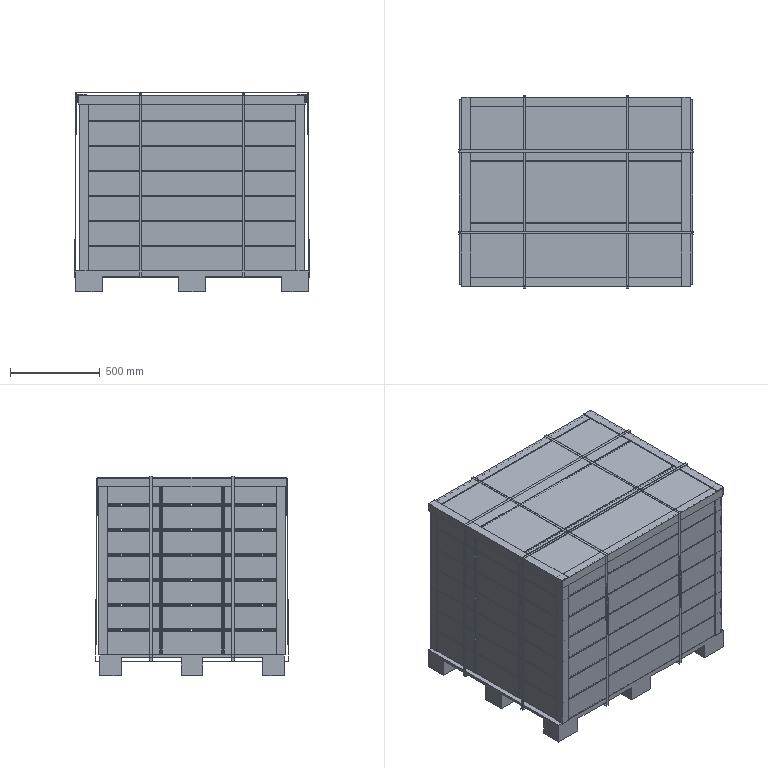Assembly | NX | mm | 34 component files | 34 solids | 431 faces | box 1307.7 x 1076.11 x 1110.92 mm | volume 176453760 mm3 | plane 419 | cylinder 12 | commonest cylinder face diameters 10 x6 6 x6
Bill of materials:
unnamed part 1 | 1 |  | Flat rectangular deck plate supported underneath by a 3x3 grid of rectangular blocks, which leaves open gaps between the blocks along both horizontal directions; the overall form resembles a pallet.
unnamed part 2 | 4 |  | Straight length of angle profile (L-shaped cross-section) with two legs that look roughly equal, cut square at both ends.
unnamed part 3 | 2 |  | Thin flat rectangular plate or sheet with no visible holes or other features; it is wider than it is tall in its main face view.
unnamed part 4 | 21 |  | Solid rectangular block or bar (a cuboid) with flat faces and sharp edges, and no visible features.
unnamed part 5 | 2 |  | Long straight angle profile (L-shaped cross-section) with legs that look roughly equal and square-cut ends, oriented horizontally.
unnamed part 6 | 2 |  | Long straight angle profile (L-shaped cross-section) with legs that look roughly equal and square-cut ends; it has the same form as the other horizontal angle but is shown in a mirrored or rotated orientation.
unnamed part 7 | 2 |  | Thin flat rectangular plate or sheet with no visible features; its face is close to square, a little taller than wide in its main face view.
Mates:
1. fix | carton 21 component
2. fix | assembly component
3. bond | carton 21 component | assembly component
4. bond | carton 20 component | assembly component
5. linear | assembly datumaxis | assembly cartesiancoordinatesystem | assembly cartesiancoordinatesystem | assembly cartesiancoordinatesystem
6. touch align | vertical_corner_protector 4 face | carton 1 face
7. touch align | vertical_corner_protector 4 face | carton 1 face
8. touch align | vertical_corner_protector 4 face | carton 20 face
9. touch align | vertical_corner_protector 3 face | carton 6 face
10. touch align | vertical_corner_protector 3 face | carton 6 face
11. touch align | vertical_corner_protector 3 face | carton 19 face
12. touch align | vertical_corner_protector 2 face | carton 6 face
13. touch align | vertical_corner_protector 2 face | carton 6 face
14. touch align | vertical_corner_protector 2 face | 103x135x10_pallet 1 face
15. touch align | vertical_corner_protector 1 face | carton 1 face
16. touch align | vertical_corner_protector 1 face | carton 1 face
17. touch align | vertical_corner_protector 1 face | 103x135x10_pallet 1 face
18. touch align | length_corner_protector 2 face | vertical_corner_protector 2 face
19. touch align | length_corner_protector 2 face | vertical_corner_protector 2 face
20. touch align | length_corner_protector 2 face | vertical_corner_protector 2 face
21. touch align | length_corner_protector 1 face | vertical_corner_protector 4 face
22. touch align | length_corner_protector 1 face | vertical_corner_protector 4 face
23. touch align | length_corner_protector 1 face | vertical_corner_protector 4 face
24. touch align | width_corner_protector 2 face | length_corner_protector 1 face
25. touch align | width_corner_protector 2 face | length_corner_protector 1 face
26. touch align | width_corner_protector 1 face | length_corner_protector 2 face
27. touch align | width_corner_protector 1 face | length_corner_protector 2 face
28. fix | assembly component
29. bond | short_packaging_strap 2 component | assembly component
30. bond | short_packaging_strap 1 component | assembly component
31. linear | assembly datumaxis | assembly cartesiancoordinatesystem | assembly cartesiancoordinatesystem
32. fix | assembly component
33. bond | long_packaging_strap 2 component | assembly component
34. bond | long_packaging_strap 1 component | assembly component
35. linear | assembly datumaxis | assembly cartesiancoordinatesystem | assembly cartesiancoordinatesystem
36. bond | carton 19 component | assembly component
37. fix | assembly component
38. bond | carton 19 component | assembly component
39. bond | carton 21 component | assembly component
40. bond | carton 20 component | assembly component
41. bond | carton 18 component | assembly component
42. bond | carton 17 component | assembly component
43. bond | carton 16 component | assembly component
44. linear | assembly datumaxis | assembly cartesiancoordinatesystem | assembly cartesiancoordinatesystem | assembly cartesiancoordinatesystem | assembly cartesiancoordinatesystem | assembly cartesiancoordinatesystem | assembly cartesiancoordinatesystem | assembly cartesiancoordinatesystem
45. linear | assembly datumaxis | assembly cartesiancoordinatesystem | assembly cartesiancoordinatesystem | assembly cartesiancoordinatesystem | assembly cartesiancoordinatesystem | assembly cartesiancoordinatesystem | assembly cartesiancoordinatesystem | assembly cartesiancoordinatesystem
46. linear | assembly datumaxis | assembly cartesiancoordinatesystem | assembly cartesiancoordinatesystem | assembly cartesiancoordinatesystem | assembly cartesiancoordinatesystem | assembly cartesiancoordinatesystem | assembly cartesiancoordinatesystem | assembly cartesiancoordinatesystem
47. bond | carton 15 component | assembly component
48. bond | carton 14 component | assembly component
49. bond | carton 13 component | assembly component
50. bond | carton 12 component | assembly component
51. bond | carton 11 component | assembly component
52. bond | carton 10 component | assembly component
53. bond | carton 9 component | assembly component
54. bond | carton 8 component | assembly component
55. bond | carton 7 component | assembly component
56. bond | carton 6 component | assembly component
57. bond | carton 5 component | assembly component
58. bond | carton 4 component | assembly component
59. bond | carton 3 component | assembly component
60. bond | carton 2 component | assembly component
61. bond | carton 1 component | assembly component
62. center | 103x135x10_pallet 1 face | 103x135x10_pallet 1 face | assembly datumplane
63. center | 103x135x10_pallet 1 face | 103x135x10_pallet 1 face | assembly datumplane
64. touch align | width_corner_protector 1 face | length_corner_protector 2 face